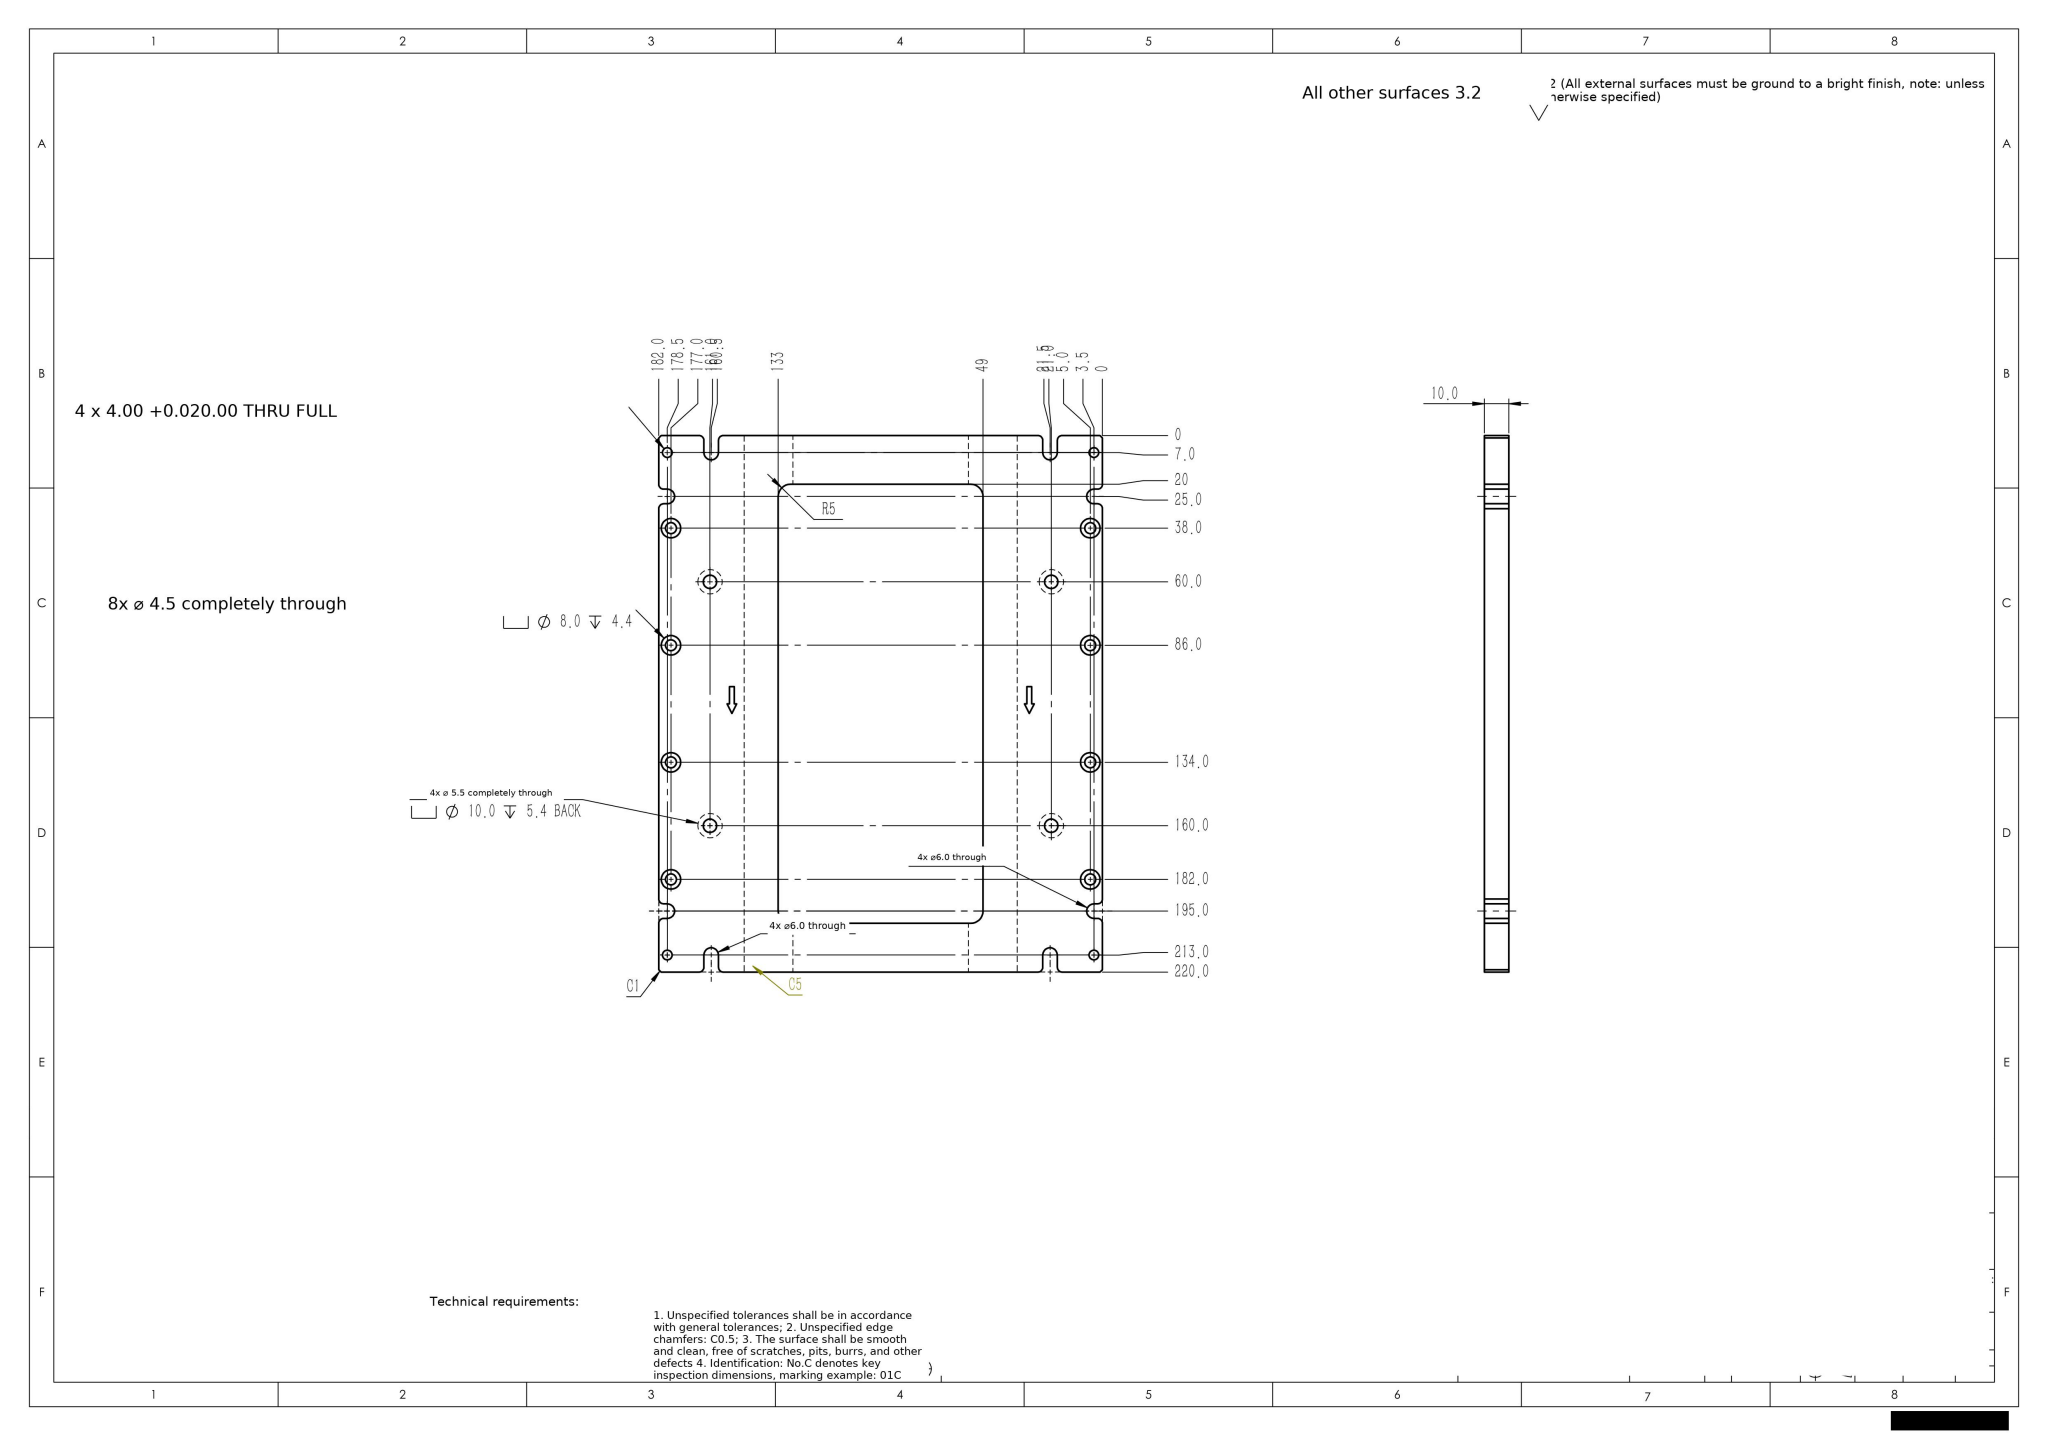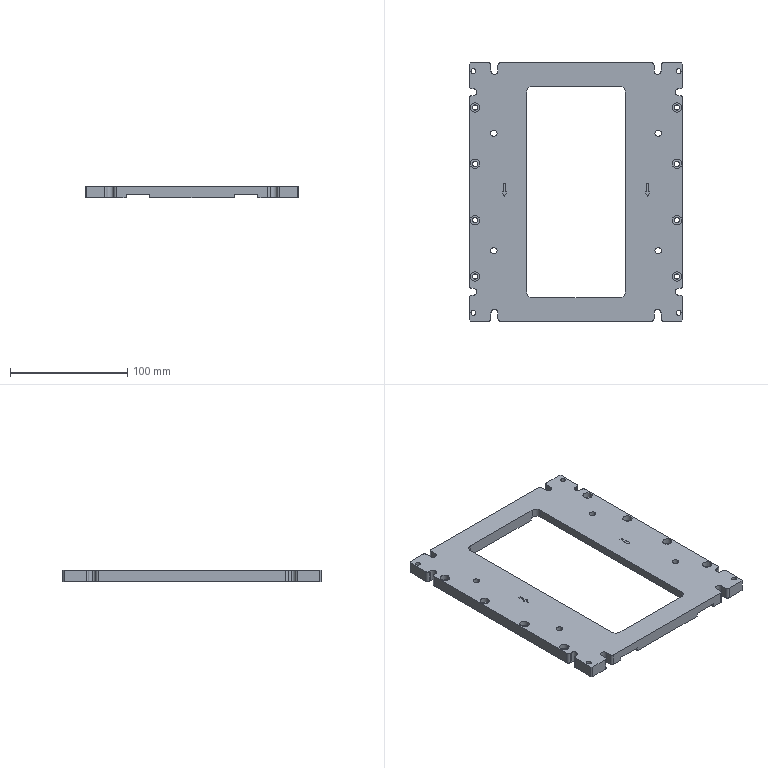Part | SolidWorks | mm | 1 solid | 163 faces | box 182 x 220 x 10 mm | volume 220482 mm3 | cylinder 86 | plane 77 | commonest cylinder face diameters 4 x24 8 x16 4.5 x16 10 x12 6 x10 5.5 x8
build123d program:
from build123d import *

# Parameters (mm, degrees)
SKETCH1_W                                       = 182
SKETCH1_H                                       = 220
BOSS_EXTRUDE1_DEPTH                             = 10
CHAMFER1_SIZE                                   = 1
SKETCH8_W                                       = 84
SKETCH8_H                                       = 30
CUT_EXTRUDE4_DEPTH                              = 144.112
FILLET1_R                                       = 5
CUT_EXTRUDE7_DEPTH                              = 144.112
M4_HEX_SOCKET_HEAD_CAP_SCREW_CBORE2_D           = 4.5
M4_HEX_SOCKET_HEAD_CAP_SCREW_CBORE2_CBORE_D     = 8
M4_HEX_SOCKET_HEAD_CAP_SCREW_CBORE2_CBORE_DEPTH = 4.4
LPATTERN1_COUNT                                 = 4
LPATTERN1_PITCH                                 = 48
LPATTERN1_COUNT_DIR2                            = 2
LPATTERN1_PITCH_DIR2                            = 172
F_4_0_4_DIAMETER_HOLE1_D                        = 4
CUT_EXTRUDE9_DEPTH                              = 144.112
M5_HEX_SOCKET_HEAD_CAP_SCREW_CBORE1_D           = 5.5
M5_HEX_SOCKET_HEAD_CAP_SCREW_CBORE1_CBORE_D     = 10
M5_HEX_SOCKET_HEAD_CAP_SCREW_CBORE1_CBORE_DEPTH = 5.4
FILLET2_R                                       = 2
SKETCH22_W                                      = 84
SKETCH22_H                                      = 20
BOSS_EXTRUDE2_DEPTH                             = 10
FILLET3_R                                       = 5
SKETCH23_W                                      = 20
SKETCH23_H                                      = 3
CUT_EXTRUDE10_DEPTH                             = 239.288
CUT_EXTRUDE11_DEPTH                             = 0.5
LPATTERN2_COUNT                                 = 2
LPATTERN2_PITCH                                 = 122


with BuildPart() as part:
    # Sketch1 → Boss-Extrude1 (new body)
    with BuildSketch(Plane.XY):
        Rectangle(SKETCH1_W, SKETCH1_H)
    extrude(amount=BOSS_EXTRUDE1_DEPTH)

    # Chamfer1
    chamfer1_edges = [part.edges().sort_by_distance(p)[0] for p in [
        (91, -110, 5),
        (-91, -110, 5),
        (-91, 110, 5),
        (91, 110, 5),
    ]]
    chamfer(chamfer1_edges, length=CHAMFER1_SIZE)

    # Sketch8 → Cut-Extrude4 (cut, through all)
    with BuildSketch(Plane.XY.offset(10)):
        with Locations((0, -95)):
            Rectangle(SKETCH8_W, SKETCH8_H)
    extrude(amount=-CUT_EXTRUDE4_DEPTH, mode=Mode.SUBTRACT)

    # Fillet1
    fillet1_edges = [part.edges().sort_by_distance(p)[0] for p in [
        (42, -80, 5),
        (-42, -80, 5),
    ]]
    fillet(fillet1_edges, radius=FILLET1_R)

    # Sketch13 → Cut-Extrude7 (cut, through all)
    with BuildSketch(Plane.XY.offset(10)):
        with BuildLine():
            Line((-37, -90), (37, -90))
            ThreePointArc((37, -90), (40.536, -88.536), (42, -85))
            Line((42, -85), (42, 85))
            ThreePointArc((42, 85), (40.536, 88.536), (37, 90))
            Line((37, 90), (-37, 90))
            ThreePointArc((-37, 90), (-40.536, 88.536), (-42, 85))
            Line((-42, 85), (-42, -85))
            ThreePointArc((-42, -85), (-40.536, -88.536), (-37, -90))
        make_face()
    extrude(amount=-CUT_EXTRUDE7_DEPTH, mode=Mode.SUBTRACT)

    # M4 Hex Socket Head Cap Screw CBORE2 (through all)
    with Locations(Plane.XY.offset(10)):
        with Locations((86, 72)):
            m4_hex_socket_head_cap_screw_cbore2 = CounterBoreHole(M4_HEX_SOCKET_HEAD_CAP_SCREW_CBORE2_D / 2, M4_HEX_SOCKET_HEAD_CAP_SCREW_CBORE2_CBORE_D / 2, M4_HEX_SOCKET_HEAD_CAP_SCREW_CBORE2_CBORE_DEPTH)

    # LPattern1: M4 Hex Socket Head Cap Screw CBORE2 4 × 2
    with Locations(*[(-j * LPATTERN1_PITCH_DIR2, -i * LPATTERN1_PITCH, 0) for i in range(LPATTERN1_COUNT) for j in range(LPATTERN1_COUNT_DIR2) if (i, j) != (0, 0)]):
        add(m4_hex_socket_head_cap_screw_cbore2, mode=Mode.SUBTRACT)

    # 4.0 _4_ Diameter Hole1 (through all)
    with Locations(Plane.XY.offset(10)):
        with Locations((-87.5, -103), (87.5, -103)):
            f_4_0_4_diameter_hole1 = Hole(F_4_0_4_DIAMETER_HOLE1_D / 2)

    # Sketch19 → Cut-Extrude9 (cut, through all)
    with BuildSketch(Plane.XY.offset(10)):
        with BuildLine():
            Line((-72.5, -110), (-72.5, -103))
            ThreePointArc((-72.5, -103), (-69.5, -100), (-66.5, -103))
            Line((-66.5, -103), (-66.5, -110))
            ThreePointArc((-66.5, -110), (-69.5, -113), (-72.5, -110))
        make_face()
        with BuildLine():
            Line((-91, -82), (-87.5, -82))
            ThreePointArc((-87.5, -82), (-84.5, -85), (-87.5, -88))
            Line((-87.5, -88), (-91, -88))
            ThreePointArc((-91, -88), (-94, -85), (-91, -82))
        make_face()
        with BuildLine():
            Line((72.5, -103), (72.5, -110))
            ThreePointArc((72.5, -110), (69.5, -113), (66.5, -110))
            Line((66.5, -110), (66.5, -103))
            ThreePointArc((66.5, -103), (69.5, -100), (72.5, -103))
        make_face()
        with BuildLine():
            Line((87.5, -82), (91, -82))
            ThreePointArc((91, -82), (94, -85), (91, -88))
            Line((91, -88), (87.5, -88))
            ThreePointArc((87.5, -88), (84.5, -85), (87.5, -82))
        make_face()
    cut_extrude9 = extrude(amount=-CUT_EXTRUDE9_DEPTH, mode=Mode.SUBTRACT)

    # Mirror4: 4.0 _4_ Diameter Hole1, Cut-Extrude9 across plane
    add(f_4_0_4_diameter_hole1.mirror(Plane.ZX), mode=Mode.SUBTRACT)
    add(cut_extrude9.mirror(Plane.ZX), mode=Mode.SUBTRACT)

    # M5 Hex Socket Head Cap Screw CBORE1 (through all)
    with Locations(Plane(origin=(0, 0, 0), x_dir=(-1, 0, 0), z_dir=(0, 0, -1))):
        with Locations((-70, 50), (70, 50), (-70, -50), (70, -50)):
            CounterBoreHole(M5_HEX_SOCKET_HEAD_CAP_SCREW_CBORE1_D / 2, M5_HEX_SOCKET_HEAD_CAP_SCREW_CBORE1_CBORE_D / 2, M5_HEX_SOCKET_HEAD_CAP_SCREW_CBORE1_CBORE_DEPTH)

    # Fillet2
    fillet2_edges = [part.edges().sort_by_distance(p)[0] for p in [
        (-66.5, -110, 5),
        (-72.5, -110, 5),
        (-91, -88, 5),
        (-91, -82, 5),
        (72.5, -110, 5),
        (66.5, -110, 5),
        (91, -82, 5),
        (91, -88, 5),
        (-72.5, 110, 5),
        (-66.5, 110, 5),
        (-91, 82, 5),
        (-91, 88, 5),
        (66.5, 110, 5),
        (72.5, 110, 5),
        (91, 88, 5),
        (91, 82, 5),
    ]]
    fillet(fillet2_edges, radius=FILLET2_R)

    # Sketch22 → Boss-Extrude2 (add)
    with BuildSketch(Plane(origin=(0, 0, 0), x_dir=(-1, 0, 0), z_dir=(0, 0, -1))):
        with Locations((0, -100)):
            Rectangle(SKETCH22_W, SKETCH22_H)
    extrude(amount=-BOSS_EXTRUDE2_DEPTH)

    # Fillet3
    fillet3_edges = [part.edges().sort_by_distance(p)[0] for p in [
        (42, -90, 5),
        (-42, -90, 5),
    ]]
    fillet(fillet3_edges, radius=FILLET3_R)

    # Sketch23 → Cut-Extrude10 (cut, through all)
    with BuildSketch(Plane.XZ.offset(110)):
        with Locations((-46, 1.5)):
            Rectangle(SKETCH23_W, SKETCH23_H)
        with Locations((46, 1.5)):
            Rectangle(SKETCH23_W, SKETCH23_H)
    extrude(amount=-CUT_EXTRUDE10_DEPTH, mode=Mode.SUBTRACT)

    # Sketch24 → Cut-Extrude11 (cut)
    with BuildSketch(Plane.XY.offset(10)):
        Polygon((62, 7), (62, 0), (63, 0), (61, -4), (59, 0), (60, 0), (60, 7), align=None)
    cut_extrude11 = extrude(amount=-CUT_EXTRUDE11_DEPTH, mode=Mode.SUBTRACT)

    # LPattern2: Cut-Extrude11 ×2
    with Locations(*[(-i * LPATTERN2_PITCH, 0, 0) for i in range(1, LPATTERN2_COUNT)]):
        add(cut_extrude11, mode=Mode.SUBTRACT)


solid = part.part